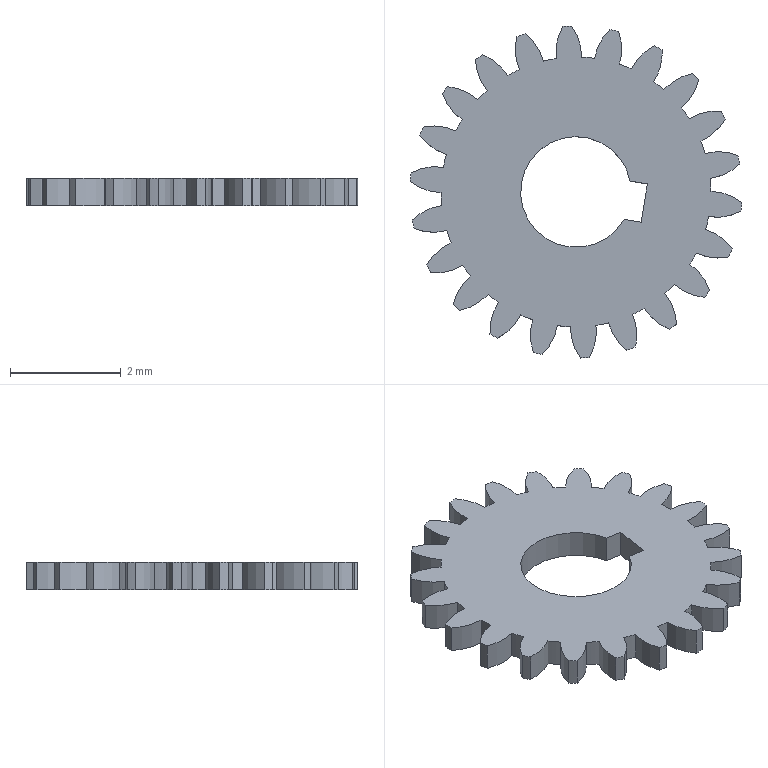Component | SolidWorks | RearAxisGear-2 | 1 solid | 99 faces | box 5.99 x 6 x 0.5 mm | volume 10 mm3 | cylinder 94 | plane 5 | commonest cylinder face diameters 1.881 x48 4.875 x22 6 x22 2 x2
build123d program:
from build123d import *

# Parameters (mm, degrees)
SKETCH1_R           = 2.438
SKETCH1_R_2         = 1
BOSS_EXTRUDE1_DEPTH = 0.5
BOSS_EXTRUDE2_START = -0.5
BOSS_EXTRUDE2_DEPTH = 0.5
CIRPATTERN1_COUNT   = 22
SKETCH3_W           = 0.5
SKETCH3_H           = 0.7
CUT_EXTRUDE1_DEPTH  = 1


with BuildPart() as part:
    # Sketch1 → Boss-Extrude1 (new body)
    with BuildSketch(Plane.XY):
        with Locations((13.57, 1.216)):
            Circle(SKETCH1_R)
        with Locations((13.57, 1.216)):
            Circle(SKETCH1_R_2, mode=Mode.SUBTRACT)
    extrude(amount=BOSS_EXTRUDE1_DEPTH)

    # Sketch2 → Boss-Extrude2 (add)
    with BuildSketch(Plane.XY.offset(0.5).offset(BOSS_EXTRUDE2_START)):
        with BuildLine():
            ThreePointArc((13.973, 3.62), (13.965, 3.92), (13.863, 4.202))
            ThreePointArc((13.863, 4.202), (13.784, 4.208), (13.705, 4.213))
            ThreePointArc((13.705, 4.213), (13.564, 3.948), (13.513, 3.653))
            ThreePointArc((13.513, 3.653), (13.744, 3.647), (13.973, 3.62))
        make_face()
    boss_extrude2 = extrude(amount=BOSS_EXTRUDE2_DEPTH)

    # CirPattern1: Boss-Extrude2 ×22 about axis
    cirpattern1_axis = Axis((13.57, 1.216, 0), (0, 0, 1))
    for i in range(1, CIRPATTERN1_COUNT):
        add(boss_extrude2.rotate(cirpattern1_axis, i * 360 / CIRPATTERN1_COUNT))

    # Sketch3 → Cut-Extrude1 (cut)
    with BuildSketch(Plane.XY):
        with Locations((14.57, 1.216)):
            Rectangle(SKETCH3_W, SKETCH3_H)
    extrude(amount=CUT_EXTRUDE1_DEPTH, mode=Mode.SUBTRACT)


solid = part.part

# Placed as in the assembly
solid = solid.moved(Location((-1.089, -2.522, 4), (0, 0, -9.237)))